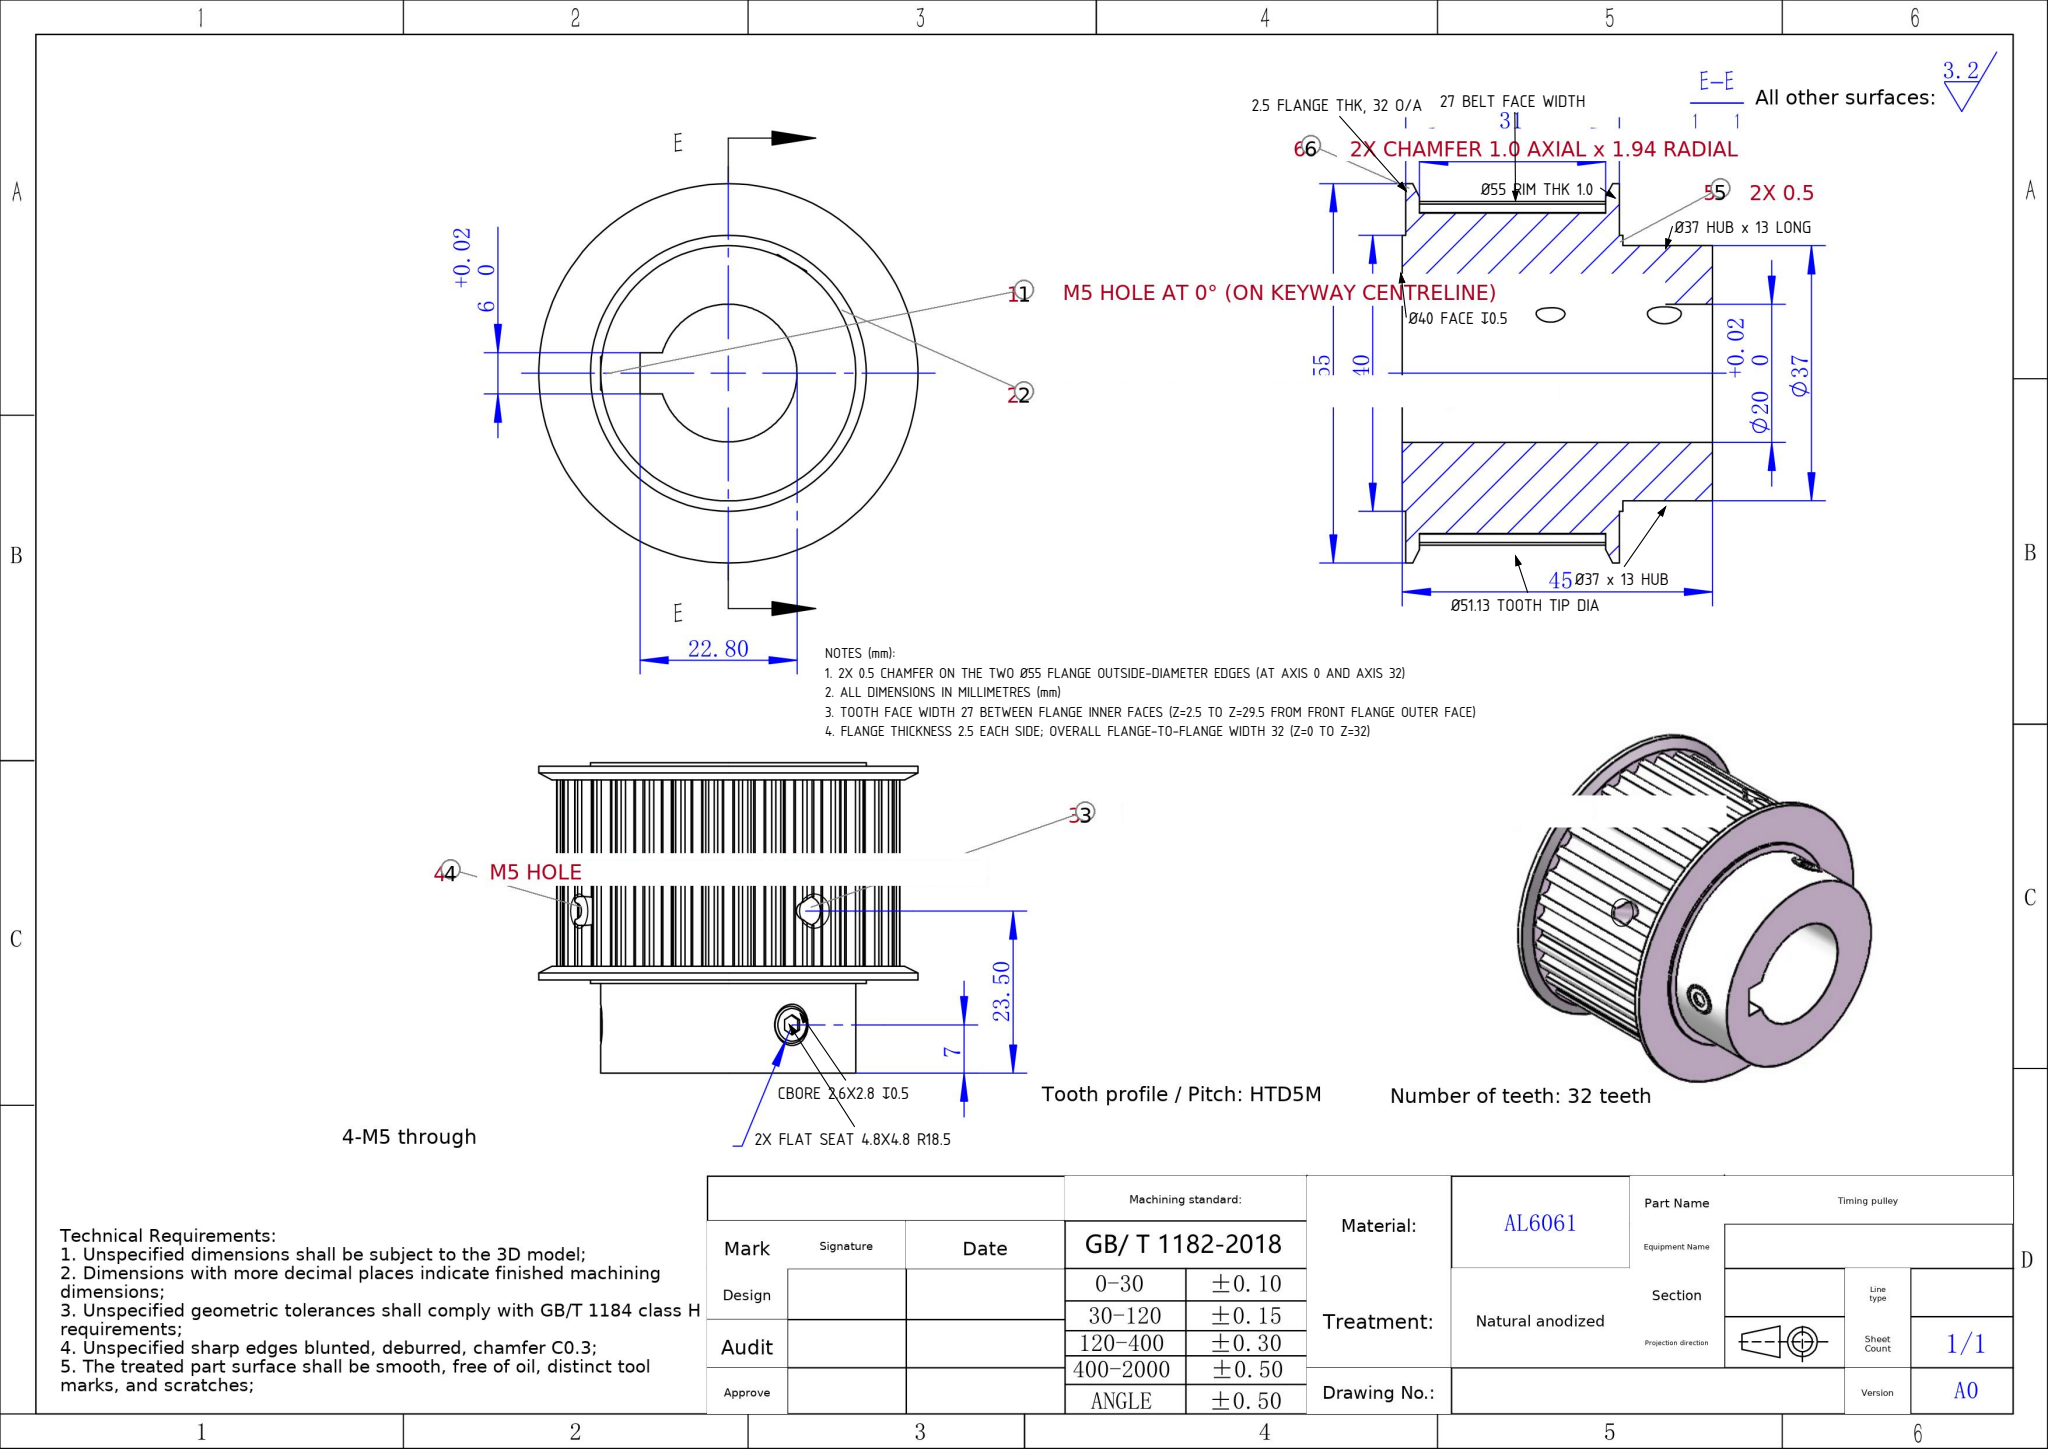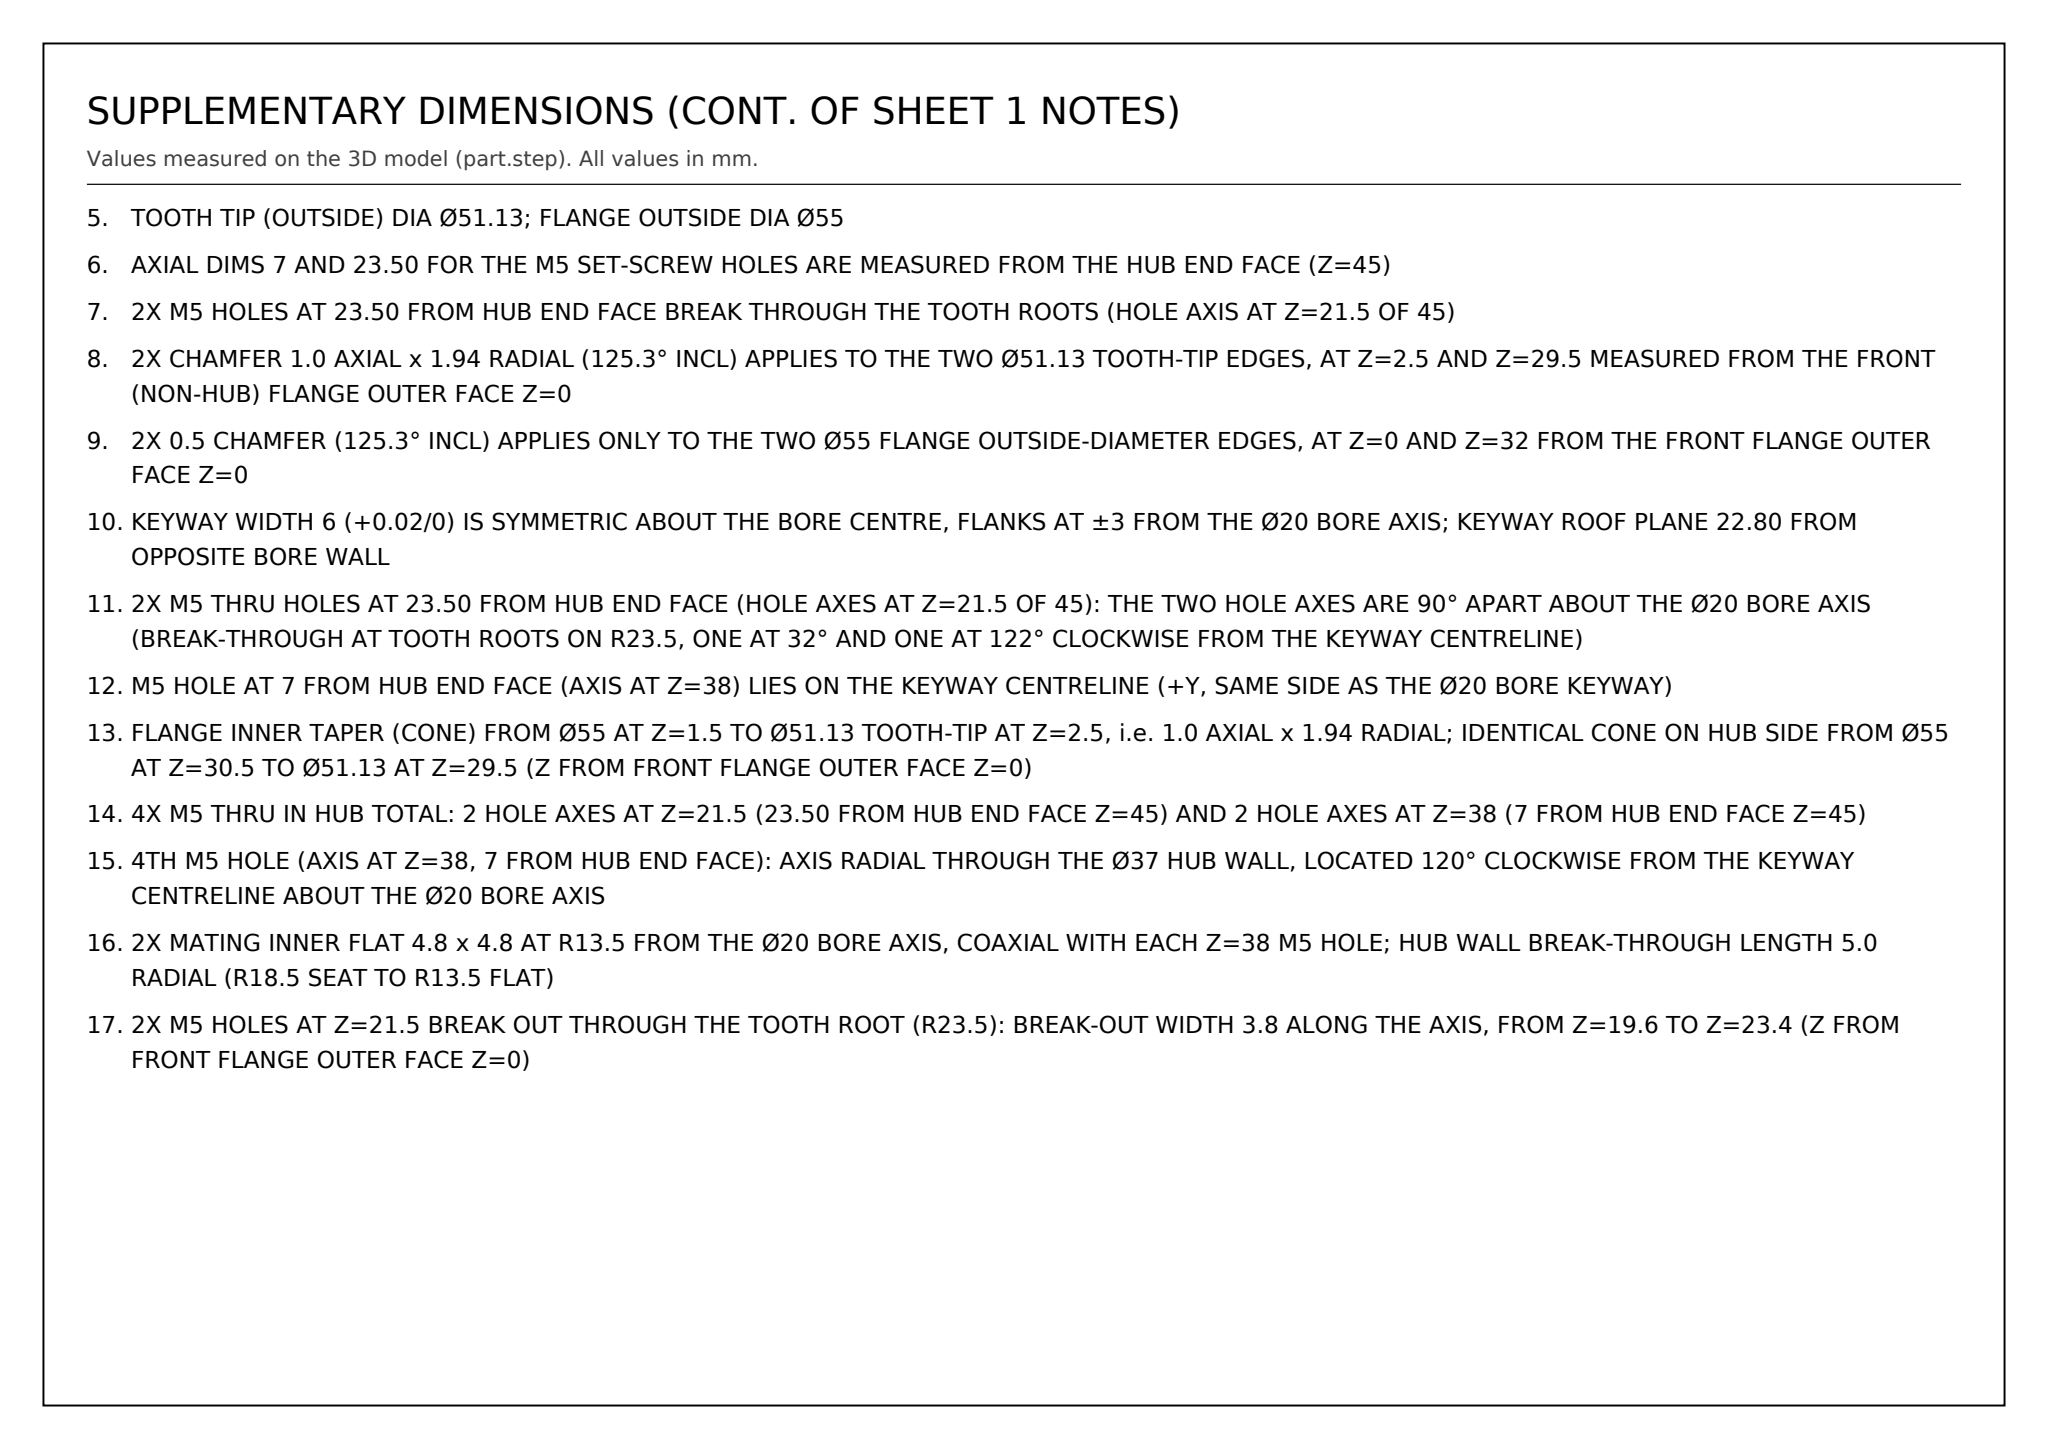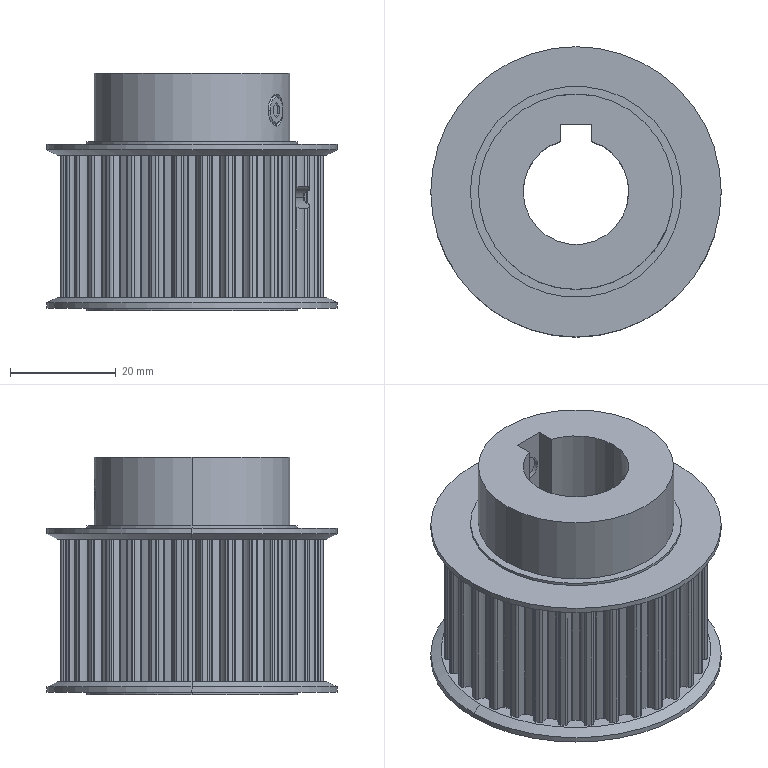Part | SolidWorks | mm | material AL6061 | 1 solid | 361 faces | box 55 x 55 x 45 mm | volume 57886 mm3 | cylinder 317 | plane 28 | cone 16 | commonest cylinder face diameters 1 x82 0.5 x76 6.55 x71 49.97 x34 46.43 x33 4.2 x4 55 x4 40 x4
Drawing notes:
BELT GROOVE (TOOTH) FACE WIDTH 27 BETWEEN THE TWO FLANGE INNER FACES (FROM 2.5 TO 29.5 ALONG THE AXIS, MEASURED FROM THE FLANGE END FACE OPPOSITE THE HUB) | from the solid: tooth-profile cylinders (dia 0.5/1.0, axis z) length 27.0; axis_planes z=2.5 and z=29.5
FLANGE THICKNESS 2.5 EACH (AXIAL); OVERALL FLANGE-TO-FLANGE WIDTH 32 (AXIS POSITIONS 0 TO 32) | from the solid: axis_planes z=0.0, 2.5, 29.5, 32.0
HUB Ø37 EXTENDS 13 FROM THE HUB-SIDE FLANGE OUTER FACE (AXIS 32) TO THE HUB END FACE (AXIS 45) | from the solid: axis_planes z=32.0 and z=45.0; bbox_xyz z=45.0
2X 0.5 CHAMFER ON THE TWO Ø55 FLANGE OUTSIDE-DIAMETER EDGES (AT AXIS 0 AND AXIS 32) | from the solid: cones [125.3 included, ref_dia 55.0, count 2]; axis_planes z=0.5 and z=31.5
TOOTH OUTSIDE (TIP) DIAMETER Ø51.13; FLANGE OUTSIDE DIAMETER Ø55 (CONCENTRIC WITH Ø20 BORE) | from the solid: cones ref_dia 51.13 and 55.0; bbox_xyz 55.0 x 55.0
ALL DIMENSIONS IN MILLIMETRES (mm) | from the solid: STEP model facts stated in mm (bbox_xyz 55.0 x 55.0 x 45.0 mm)
TOOTH FACE WIDTH 27 BETWEEN FLANGE INNER FACES (Z=2.5 TO Z=29.5 FROM FRONT FLANGE OUTER FACE) | from the solid: axis_planes z=2.5 and z=29.5; tooth-root cylinders length 27.0
FLANGE THICKNESS 2.5 EACH SIDE; OVERALL FLANGE-TO-FLANGE WIDTH 32 (Z=0 TO Z=32) | from the solid: axis_planes z=0.0, 2.5, 29.5, 32.0
HUB Ø37 x 13 LONG, FROM REAR FLANGE FACE (Z=32) TO HUB END FACE (Z=45) | from the solid: axis_planes z=32.0 and z=45.0; bbox_xyz z=45
TOOTH TIP (OUTSIDE) DIA Ø51.13; FLANGE OUTSIDE DIA Ø55 | from the solid: cones [125.3, 51.13] and [125.3, 55.0]; bbox_xyz x,y = 55
AXIAL DIMS 7 AND 23.50 FOR THE M5 SET-SCREW HOLES ARE MEASURED FROM THE HUB END FACE (Z=45) | from the solid: tooth-root cylinders at [39.96,47.38] and [47.38,15.04] split into 17.06 + 6.06 segments, gap centred at z=21.5 = 23.5 from z=45
2X M5 HOLES AT 23.50 FROM HUB END FACE BREAK THROUGH THE TOOTH ROOTS (HOLE AXIS AT Z=21.5 OF 45) | from the solid: tooth-root cylinders length 27 interrupted into 17.06 and 6.06 segments at two circumferential locations
2X CHAMFER 1.0 AXIAL x 1.94 RADIAL (125.3° INCL) APPLIES TO THE TWO Ø51.13 TOOTH-TIP EDGES, AT Z=2.5 AND Z=29.5 MEASURED FROM THE FRONT (NON-HUB) FLANGE OUTER FACE Z=0 | from the solid: cones[included_angle,ref_dia]: [125.3, 51.13] qty 2; axis_planes z=2.5 and z=29.5
2X 0.5 CHAMFER (125.3° INCL) APPLIES ONLY TO THE TWO Ø55 FLANGE OUTSIDE-DIAMETER EDGES, AT Z=0 AND Z=32 FROM THE FRONT FLANGE OUTER FACE Z=0 | from the solid: cones[included_angle,ref_dia]: [125.3, 55.0] qty 2; axis_planes z=0.0/0.5 and z=31.5/32.0
KEYWAY WIDTH 6 (+0.02/0) IS SYMMETRIC ABOUT THE BORE CENTRE, FLANKS AT ±3 FROM THE Ø20 BORE AXIS; KEYWAY ROOF PLANE 22.80 FROM OPPOSITE BORE WALL | from the solid: axis_planes x=24.5 and x=30.5 (6 apart, bore axis x=27.5); axis_plane y=40.3 (=17.5+22.80)
2X M5 THRU HOLES AT 23.50 FROM HUB END FACE (HOLE AXES AT Z=21.5 OF 45): THE TWO HOLE AXES ARE 90° APART ABOUT THE Ø20 BORE AXIS (BREAK-THROUGH AT TOOTH ROOTS ON R23.5, ONE AT 32° AND ONE AT 122° CLOCKWISE FROM THE KEYWAY CENTRELINE) | from the solid: cylinders: root-fillet arcs Ø0.5 at (40.0,47.4) and (47.4,15.0) each interrupted from z=19.6 to z=23.4 (hole break-through); both centres at R23.5 from bore axis (27.5,27.5), angular positions 57.9° and -32.1° i.e. exactly 90° apart; keyway roof plane y=40.3 fixes keyway centreline at +Y (90°)
M5 HOLE AT 7 FROM HUB END FACE (AXIS AT Z=38) LIES ON THE KEYWAY CENTRELINE (+Y, SAME SIDE AS THE Ø20 BORE KEYWAY) | from the solid: axis_planes y=45.5 and y=46.0 (socket/counterbore faces) centred at x=27.5, z=36.6-40.4 i.e. z centre 38 = 45-7, on the +Y side matching keyway roof plane y=40.3 (x 24.5 to 30.5)
FLANGE RIM Ø55 AXIAL THICKNESS 1.0 EACH SIDE: Z=0.5 TO Z=1.5 AND Z=30.5 TO Z=31.5, MEASURED FROM FRONT (NON-HUB) FLANGE OUTER FACE Z=0 | from the solid: cylinders: boss/shaft dia 55.0 axis z from 0.5 to 1.5; dia 55.0 axis z from 30.5 to 31.5
Ø40 RECESSED FACE 0.5 DEEP AT EACH FLANGE OUTER FACE: Ø40 BAND Z=0 TO Z=0.5 (FRONT) AND Z=31.5 TO Z=32 (HUB SIDE), GIVING THE 0.5 AXIAL STEP BETWEEN THE Ø40 FACES AND THE Ø55 RIM FACES | from the solid: cylinders: dia 40.0 axis z from 0.0 to 0.5 and from 31.5 to 32.0; planes z=0.0 and z=32.0 extent x,y 7.5-47.5 (Ø40)
FLANGE INNER TAPER (CONE) FROM Ø55 AT Z=1.5 TO Ø51.13 TOOTH-TIP AT Z=2.5, i.e. 1.0 AXIAL x 1.94 RADIAL; IDENTICAL CONE ON HUB SIDE FROM Ø55 AT Z=30.5 TO Ø51.13 AT Z=29.5 (Z FROM FRONT FLANGE OUTER FACE Z=0) | from the solid: dia 55.0 cylinders end at z=1.5 and z=30.5; planes z=2.5 and z=29.5 extent x,y 1.9-53.1 (Ø51.2 tooth-tip face)
4X M5 THRU IN HUB TOTAL: 2 HOLE AXES AT Z=21.5 (23.50 FROM HUB END FACE Z=45) AND 2 HOLE AXES AT Z=38 (7 FROM HUB END FACE Z=45) | from the solid: Pairs of radial flats/recesses at z=35.6-40.4 (planes y=46.0, y=45.5, y=41.0 and inclined planes bbox_from [38.0,18.7,35.6] / [42.3,16.2,35.6]); tooth-root arc breaks at z=19.6-23.4
4TH M5 HOLE (AXIS AT Z=38, 7 FROM HUB END FACE): AXIS RADIAL THROUGH THE Ø37 HUB WALL, LOCATED 120° CLOCKWISE FROM THE KEYWAY CENTRELINE ABOUT THE Ø20 BORE AXIS | from the solid: Inclined plane bbox_from [42.3,16.2,35.6] size [2.4,4.1,4.8], angles 30°/60°/90° to X/Y/Z; its face centre (43.5,18.25) lies at R18.5 and -30° from +X, i.e. 120° CW from the +Y keyway centreline
2X FLAT SEAT (SPOTFACE) 4.8 x 4.8 MILLED TANGENT TO THE Ø37 HUB OD, SEAT FACE AT R18.5 FROM THE Ø20 BORE AXIS, CENTRED ON THE TWO M5 HOLE AXES AT Z=38 (ONE ON THE KEYWAY CENTRELINE, ONE AT 120° CW) | from the solid: Plane y=46.0 extent x 25.1-29.9, z 35.6-40.4 (R18.5 from axis 27.5,27.5); matching inclined plane at R18.5, bbox_from [42.3,16.2,35.6] size [2.4,4.1,4.8]
2X RECESS (COUNTERBORE) 0.5 DEEP AT EACH Z=38 M5 HOLE ENTRY: FLOOR 2.6 x 2.8 AT R18.0 FROM THE Ø20 BORE AXIS, 0.5 BELOW THE R18.5 FLAT SEAT | from the solid: Plane y=45.5 extent x 26.2-28.8, z 36.6-39.4, area 5; side walls planes x=26.2 and x=28.8 extent y 45.5-46.0, z 37.3-38.7
2X MATING INNER FLAT 4.8 x 4.8 AT R13.5 FROM THE Ø20 BORE AXIS, COAXIAL WITH EACH Z=38 M5 HOLE; HUB WALL BREAK-THROUGH LENGTH 5.0 RADIAL (R18.5 SEAT TO R13.5 FLAT) | from the solid: Plane y=41.0 extent x 25.1-29.9, z 35.6-40.4 (R13.5 from axis); inclined plane bbox_from [38.0,18.7,35.6] size [2.4,4.1,4.8] with face at R13.5
2X M5 HOLES AT Z=21.5 BREAK OUT THROUGH THE TOOTH ROOT (R23.5): BREAK-OUT WIDTH 3.8 ALONG THE AXIS, FROM Z=19.6 TO Z=23.4 (Z FROM FRONT FLANGE OUTER FACE Z=0) | from the solid: Tooth-root fillet arcs R0.25 at (40.0,47.4) and (47.4,15.0) are interrupted: segments z 2.5-19.6 and z 23.4-29.5